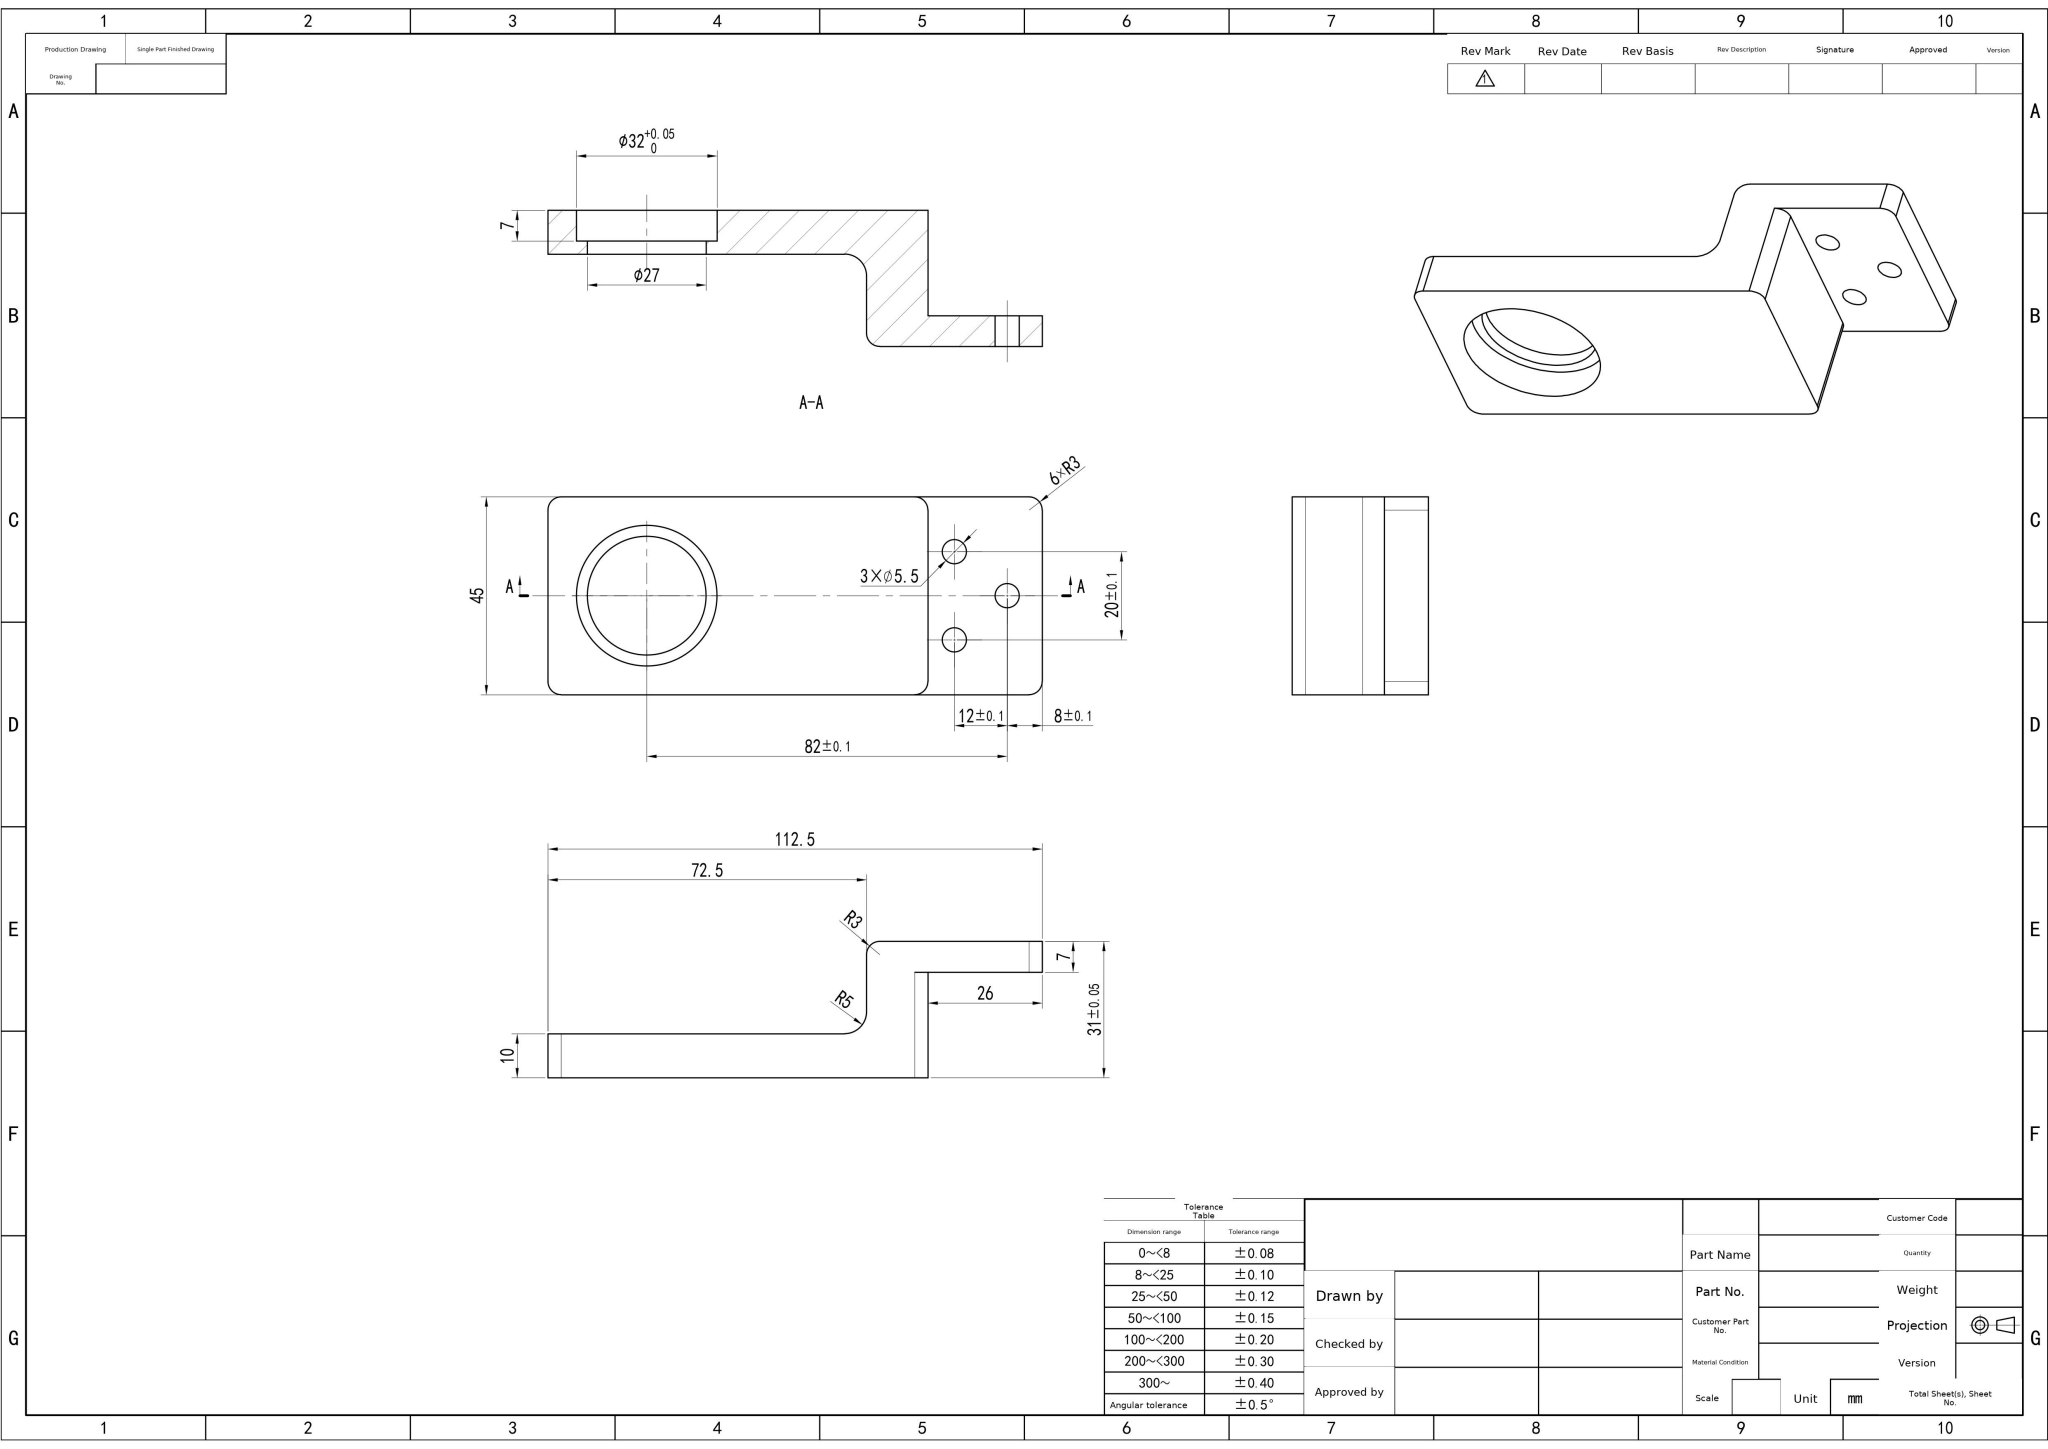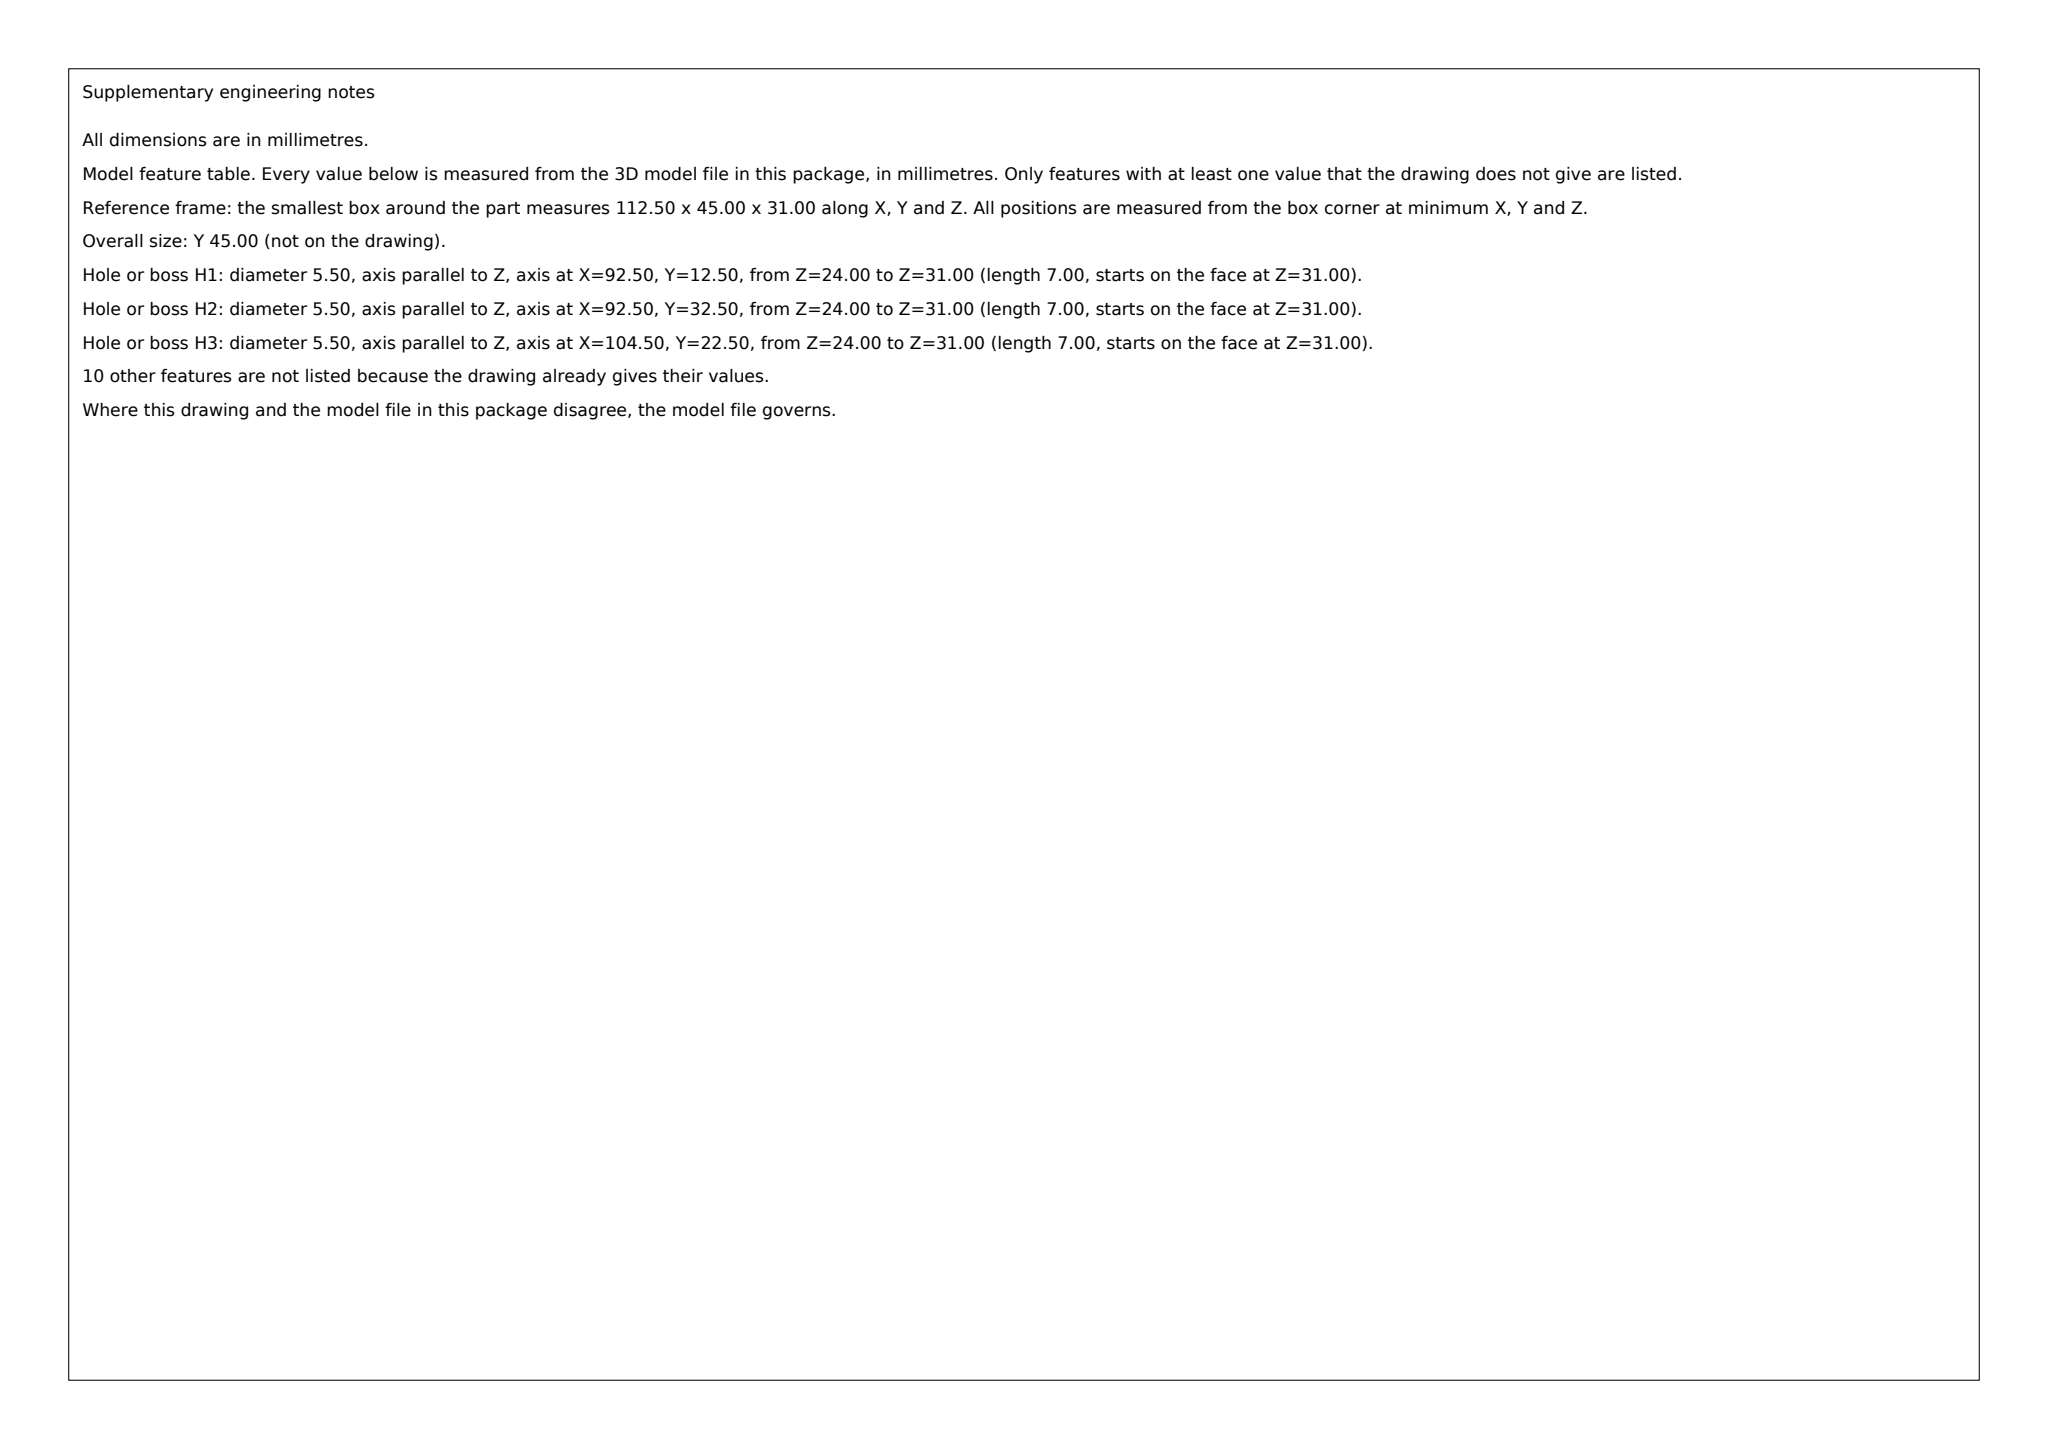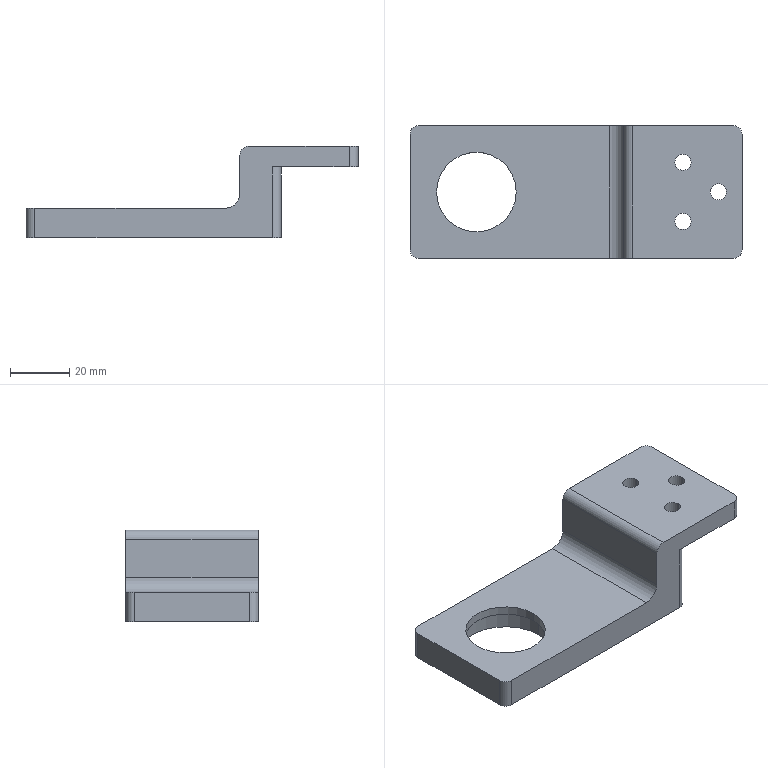Part | SolidWorks | mm | 1 solid | 29 faces | box 112.5 x 45 x 31 mm | volume 52495 mm3 | cylinder 18 | plane 11 | commonest cylinder face diameters 6 x7 5.5 x6 32 x2 27 x2 10 x1